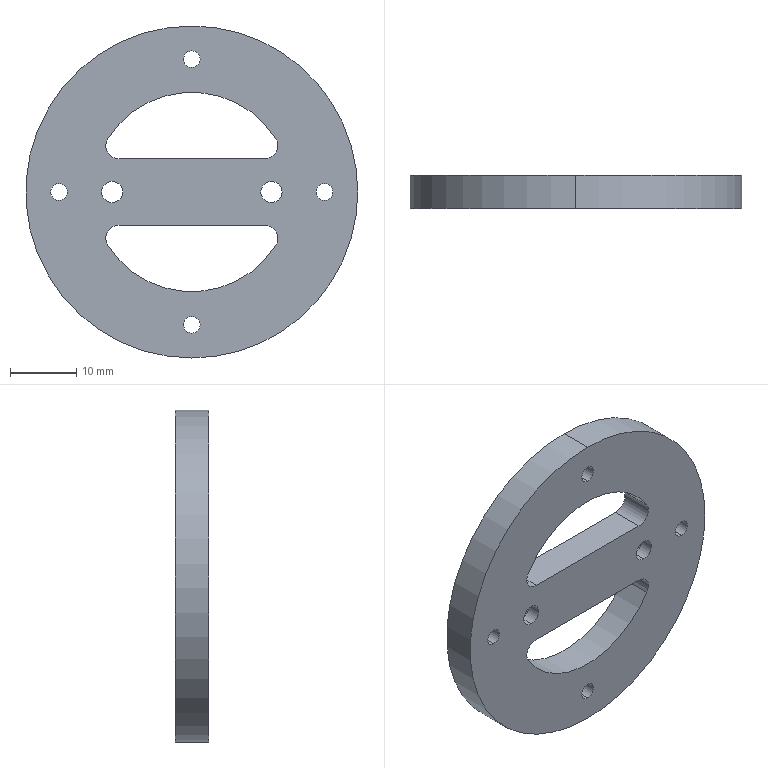CAM job | Mastercam | mm | 6 operations | part box 50 x 5 x 50
1. Contour (Ramp) | 4 - 4 平铣刀
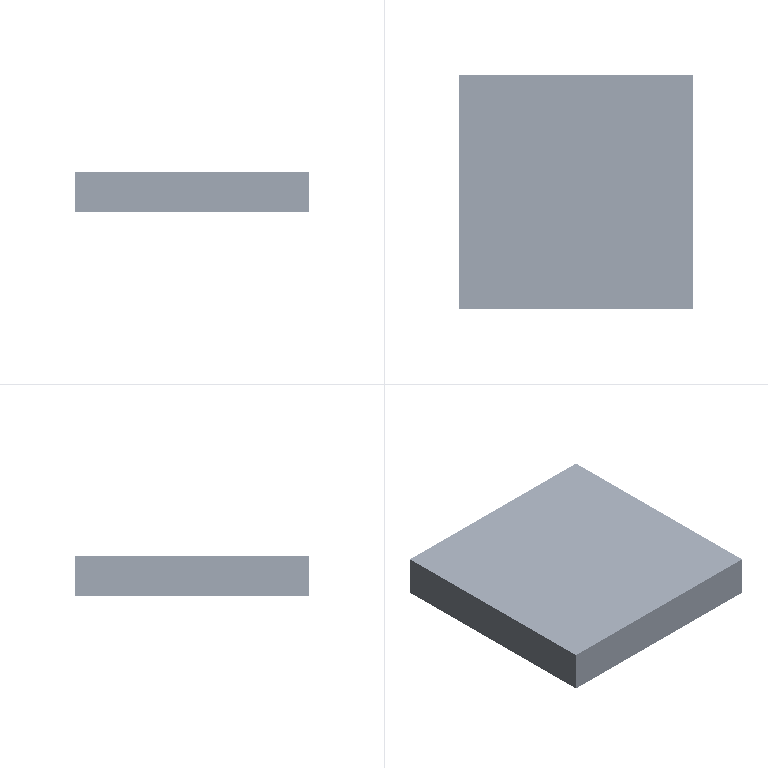2. Contour (2D) | 4 - 4 平铣刀
3. Contour (Ramp) | 4 - 4 平铣刀
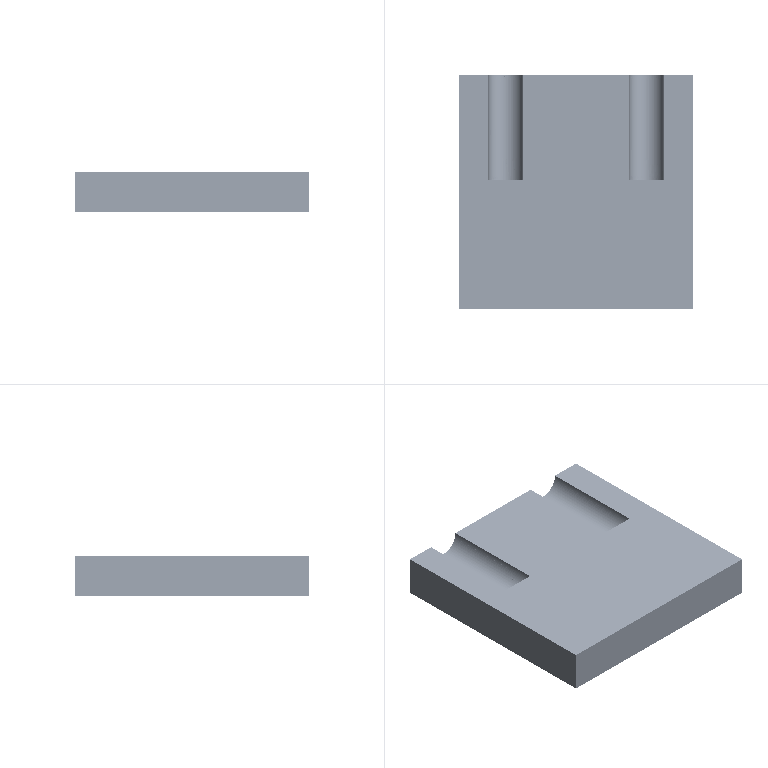4. Contour (2D) | 4 - 4 平铣刀
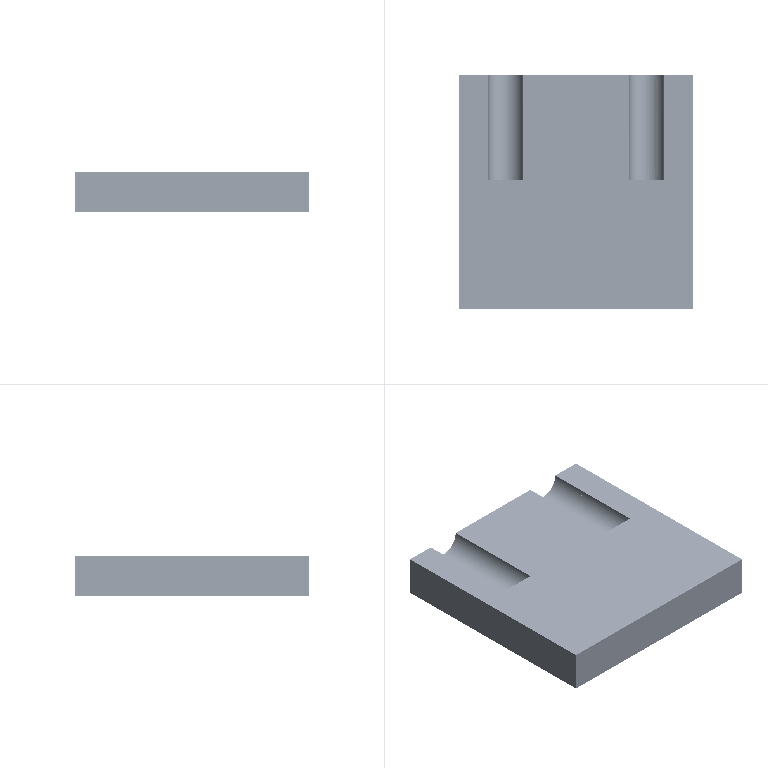5. Drill/Counterbore | 7 - 4 倒角刀
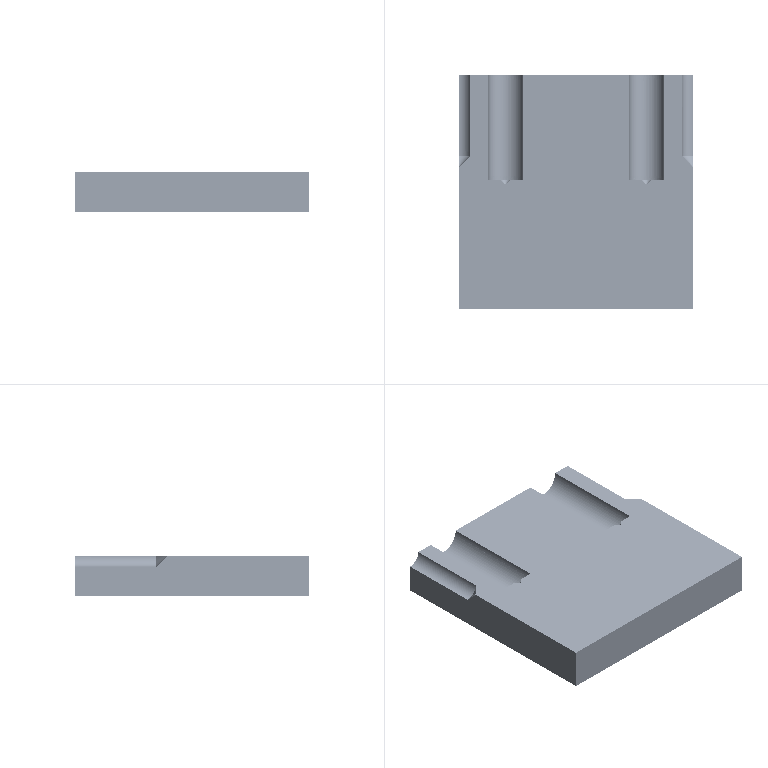6. Contour (2D chamfer) | 7 - 4 倒角刀